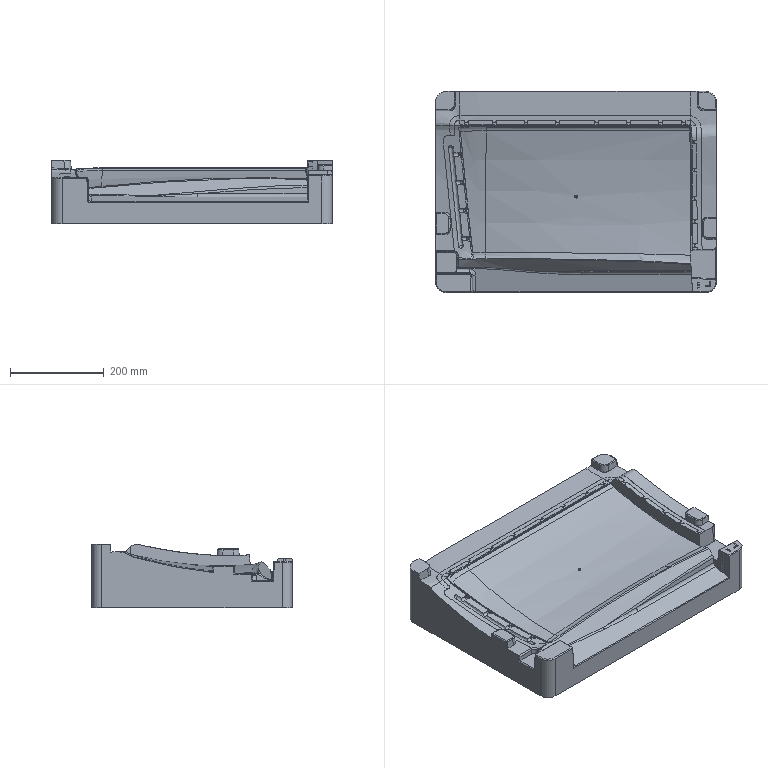CAM job | NX | mm | 3-axis | 1 set-up | 2 operations | part box 599.5 x 429.5 x 136
set-up 1
1. Cavity Milling | Mill Mill5 D63R6 | CAVITY_MILL | path 1006651.343 mm | 330.971 min
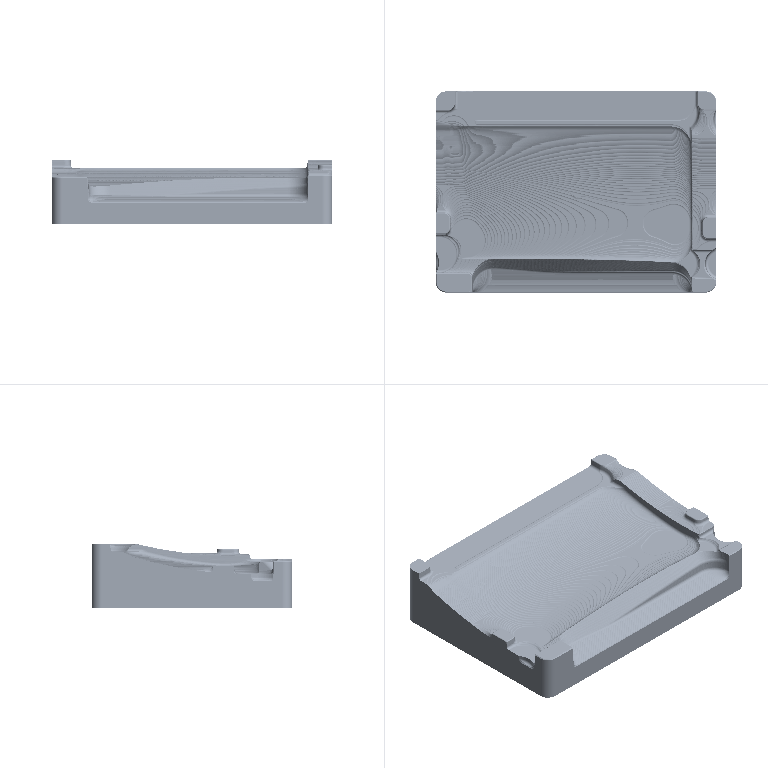2. Cavity Milling | Mill Mill5 D63R6 | CAVITY_MILL_COPY | path 914805.701 mm | 302.579 min